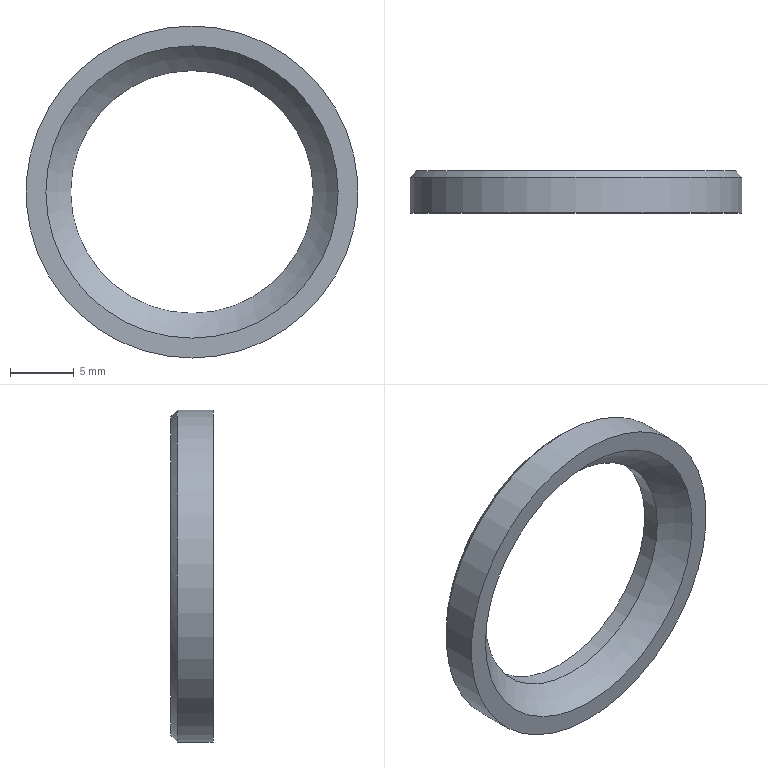Component | NX | SEAL_RING | 1 solid | 6 faces | box 26 x 3.3 x 26 mm | volume 681 mm3 | plane 2 | cylinder 2 | sphere 1 | cone 1 | commonest cylinder face diameters 19 x1 26 x1
STEP:
#1=CARTESIAN_POINT('',(0.,0.,0.));
#2=DIRECTION('',(0.,0.,1.));
#3=DIRECTION('',(1.,0.,0.));
#4=AXIS2_PLACEMENT_3D('',#1,#2,#3);
#5=CARTESIAN_POINT('',(0.,27.432,31.5));
#6=VERTEX_POINT('',#5);
#7=CARTESIAN_POINT('',(0.,27.432,19.));
#8=DIRECTION('',(0.,1.,0.));
#9=DIRECTION('',(0.,0.,1.));
#10=AXIS2_PLACEMENT_3D('',#7,#8,#9);
#11=CIRCLE('',#10,12.5);
#12=CARTESIAN_POINT('',(0.,27.432,32.));
#13=DIRECTION('',(0.,-1.,0.));
#14=DIRECTION('',(0.,0.,1.));
#15=AXIS2_PLACEMENT_3D('',#12,#13,#14);
#16=PLANE('',#15);
#17=CARTESIAN_POINT('',(-0.5,0.));
#18=CARTESIAN_POINT('',(-0.5,-21.651));
#19=CARTESIAN_POINT('',(-19.25,-10.825));
#20=CARTESIAN_POINT('',(-38.,-0.));
#21=CARTESIAN_POINT('',(-19.25,10.825));
#22=CARTESIAN_POINT('',(-0.5,21.651));
#23=CARTESIAN_POINT('',(-0.5,0.));
#24=(BOUNDED_CURVE()B_SPLINE_CURVE(2,(#17,#18,#19,#20,#21,#22,#23),.UNSPECIFIED.,.T.,.F.)B_SPLINE_CURVE_WITH_KNOTS((1,2,2,2,2,1),(-2.094,0.,2.094,4.189,6.283,8.378),.UNSPECIFIED.)CURVE()GEOMETRIC_REPRESENTATION_ITEM()RATIONAL_B_SPLINE_CURVE((1.,0.5,1.,0.5,1.,0.5,1.))REPRESENTATION_ITEM(''));
#25=(GEOMETRIC_REPRESENTATION_CONTEXT(2)PARAMETRIC_REPRESENTATION_CONTEXT()REPRESENTATION_CONTEXT('',''));
#26=DEFINITIONAL_REPRESENTATION('',(#24),#25);
#27=PCURVE('',#16,#26);
#28=CARTESIAN_POINT('',(0.,27.432,19.));
#29=DIRECTION('',(0.,-1.,0.));
#30=DIRECTION('',(0.,0.,1.));
#31=AXIS2_PLACEMENT_3D('',#28,#29,#30);
#32=CONICAL_SURFACE('',#31,12.5,0.7854);
#33=CARTESIAN_POINT('',(6.283,0.));
#34=DIRECTION('',(-1.,0.));
#35=VECTOR('',#34,1.);
#36=LINE('',#33,#35);
#37=(GEOMETRIC_REPRESENTATION_CONTEXT(2)PARAMETRIC_REPRESENTATION_CONTEXT()REPRESENTATION_CONTEXT('',''));
#38=DEFINITIONAL_REPRESENTATION('',(#36),#37);
#39=PCURVE('',#32,#38);
#40=SURFACE_CURVE('',#11,(#27,#39),.PCURVE_S1.);
#41=EDGE_CURVE('',#6,#6,#40,.T.);
#42=ORIENTED_EDGE('',*,*,#41,.T.);
#43=EDGE_LOOP('',(#42));
#44=FACE_BOUND('',#43,.T.);
#45=CARTESIAN_POINT('',(0.,27.432,9.5));
#46=VERTEX_POINT('',#45);
#47=CARTESIAN_POINT('',(0.,27.432,19.));
#48=DIRECTION('',(0.,1.,0.));
#49=DIRECTION('',(0.,0.,-1.));
#50=AXIS2_PLACEMENT_3D('',#47,#48,#49);
#51=CIRCLE('',#50,9.5);
#52=CARTESIAN_POINT('',(-22.5,0.));
#53=CARTESIAN_POINT('',(-22.5,16.454));
#54=CARTESIAN_POINT('',(-8.25,8.227));
#55=CARTESIAN_POINT('',(6.,0.));
#56=CARTESIAN_POINT('',(-8.25,-8.227));
#57=CARTESIAN_POINT('',(-22.5,-16.454));
#58=CARTESIAN_POINT('',(-22.5,0.));
#59=(BOUNDED_CURVE()B_SPLINE_CURVE(2,(#52,#53,#54,#55,#56,#57,#58),.UNSPECIFIED.,.T.,.F.)B_SPLINE_CURVE_WITH_KNOTS((1,2,2,2,2,1),(-2.094,0.,2.094,4.189,6.283,8.378),.UNSPECIFIED.)CURVE()GEOMETRIC_REPRESENTATION_ITEM()RATIONAL_B_SPLINE_CURVE((1.,0.5,1.,0.5,1.,0.5,1.))REPRESENTATION_ITEM(''));
#60=(GEOMETRIC_REPRESENTATION_CONTEXT(2)PARAMETRIC_REPRESENTATION_CONTEXT()REPRESENTATION_CONTEXT('',''));
#61=DEFINITIONAL_REPRESENTATION('',(#59),#60);
#62=PCURVE('',#16,#61);
#63=CARTESIAN_POINT('',(0.,27.432,19.));
#64=DIRECTION('',(0.,1.,0.));
#65=DIRECTION('',(0.,0.,-1.));
#66=AXIS2_PLACEMENT_3D('',#63,#64,#65);
#67=CYLINDRICAL_SURFACE('',#66,9.5);
#68=CARTESIAN_POINT('',(0.,0.));
#69=DIRECTION('',(1.,0.));
#70=VECTOR('',#69,1.);
#71=LINE('',#68,#70);
#72=(GEOMETRIC_REPRESENTATION_CONTEXT(2)PARAMETRIC_REPRESENTATION_CONTEXT()REPRESENTATION_CONTEXT('',''));
#73=DEFINITIONAL_REPRESENTATION('',(#71),#72);
#74=PCURVE('',#67,#73);
#75=SURFACE_CURVE('',#51,(#62,#74),.PCURVE_S1.);
#76=EDGE_CURVE('',#46,#46,#75,.T.);
#77=ORIENTED_EDGE('',*,*,#76,.F.);
#78=EDGE_LOOP('',(#77));
#79=FACE_BOUND('',#78,.T.);
#80=ADVANCED_FACE('',(#44,#79),#16,.F.);
#81=CARTESIAN_POINT('',(0.,26.04,9.5));
#82=VERTEX_POINT('',#81);
#83=CARTESIAN_POINT('',(0.,26.04,19.));
#84=DIRECTION('',(0.,1.,0.));
#85=DIRECTION('',(0.,0.,-1.));
#86=AXIS2_PLACEMENT_3D('',#83,#84,#85);
#87=CIRCLE('',#86,9.5);
#88=CARTESIAN_POINT('',(0.,-1.392));
#89=DIRECTION('',(1.,0.));
#90=VECTOR('',#89,1.);
#91=LINE('',#88,#90);
#92=(GEOMETRIC_REPRESENTATION_CONTEXT(2)PARAMETRIC_REPRESENTATION_CONTEXT()REPRESENTATION_CONTEXT('',''));
#93=DEFINITIONAL_REPRESENTATION('',(#91),#92);
#94=PCURVE('',#67,#93);
#95=CARTESIAN_POINT('',(0.,14.432,19.));
#96=DIRECTION('',(0.,1.,0.));
#97=DIRECTION('',(0.,0.,1.));
#98=AXIS2_PLACEMENT_3D('',#95,#96,#97);
#99=SPHERICAL_SURFACE('',#98,15.);
#100=CARTESIAN_POINT('',(3.142,0.8849));
#101=CARTESIAN_POINT('',(3.237,0.8849));
#102=CARTESIAN_POINT('',(3.427,0.8849));
#103=CARTESIAN_POINT('',(3.713,0.8849));
#104=CARTESIAN_POINT('',(3.998,0.8849));
#105=CARTESIAN_POINT('',(4.284,0.8849));
#106=CARTESIAN_POINT('',(4.57,0.8849));
#107=CARTESIAN_POINT('',(4.855,0.8849));
#108=CARTESIAN_POINT('',(5.141,0.8849));
#109=CARTESIAN_POINT('',(5.426,0.8849));
#110=CARTESIAN_POINT('',(5.712,0.8849));
#111=CARTESIAN_POINT('',(5.998,0.8849));
#112=CARTESIAN_POINT('',(6.283,0.8849));
#113=CARTESIAN_POINT('',(6.569,0.8849));
#114=CARTESIAN_POINT('',(6.854,0.8849));
#115=CARTESIAN_POINT('',(7.14,0.8849));
#116=CARTESIAN_POINT('',(7.426,0.8849));
#117=CARTESIAN_POINT('',(7.711,0.8849));
#118=CARTESIAN_POINT('',(7.997,0.8849));
#119=CARTESIAN_POINT('',(8.282,0.8849));
#120=CARTESIAN_POINT('',(8.568,0.8849));
#121=CARTESIAN_POINT('',(8.854,0.8849));
#122=CARTESIAN_POINT('',(9.139,0.8849));
#123=CARTESIAN_POINT('',(9.33,0.8849));
#124=CARTESIAN_POINT('',(9.425,0.8849));
#125=B_SPLINE_CURVE_WITH_KNOTS('',3,(#100,#101,#102,#103,#104,#105,#106,#107,#108,#109,#110,#111,#112,#113,#114,#115,#116,#117,#118,#119,#120,#121,#122,#123,#124),.UNSPECIFIED.,.F.,.F.,(4,1,1,1,1,1,1,1,1,1,1,1,1,1,1,1,1,1,1,1,1,1,4),(0.,0.2856,0.5712,0.8568,1.142,1.428,1.714,1.999,2.285,2.57,2.856,3.142,3.427,3.713,3.998,4.284,4.57,4.855,5.141,5.426,5.712,5.998,6.283),.QUASI_UNIFORM_KNOTS.);
#126=(GEOMETRIC_REPRESENTATION_CONTEXT(2)PARAMETRIC_REPRESENTATION_CONTEXT()REPRESENTATION_CONTEXT('',''));
#127=DEFINITIONAL_REPRESENTATION('',(#125),#126);
#128=PCURVE('',#99,#127);
#129=SURFACE_CURVE('',#87,(#94,#128),.PCURVE_S1.);
#130=EDGE_CURVE('',#82,#82,#129,.T.);
#131=ORIENTED_EDGE('',*,*,#130,.T.);
#132=CARTESIAN_POINT('',(0.,26.04,9.5));
#133=CARTESIAN_POINT('',(0.,27.432,9.5));
#134=B_SPLINE_CURVE_WITH_KNOTS('',1,(#132,#133),.UNSPECIFIED.,.F.,.F.,(2,2),(-1.392,0.),.PIECEWISE_BEZIER_KNOTS.);
#135=CARTESIAN_POINT('',(6.283,0.));
#136=DIRECTION('',(0.,1.));
#137=VECTOR('',#136,1.);
#138=LINE('',#135,#137);
#139=(GEOMETRIC_REPRESENTATION_CONTEXT(2)PARAMETRIC_REPRESENTATION_CONTEXT()REPRESENTATION_CONTEXT('',''));
#140=DEFINITIONAL_REPRESENTATION('',(#138),#139);
#141=PCURVE('',#67,#140);
#142=CARTESIAN_POINT('',(0.,0.));
#143=DIRECTION('',(0.,1.));
#144=VECTOR('',#143,1.);
#145=LINE('',#142,#144);
#146=(GEOMETRIC_REPRESENTATION_CONTEXT(2)PARAMETRIC_REPRESENTATION_CONTEXT()REPRESENTATION_CONTEXT('',''));
#147=DEFINITIONAL_REPRESENTATION('',(#145),#146);
#148=PCURVE('',#67,#147);
#149=SEAM_CURVE('',#134,(#141,#148),.PCURVE_S1.);
#150=EDGE_CURVE('',#82,#46,#149,.T.);
#151=ORIENTED_EDGE('',*,*,#150,.T.);
#152=ORIENTED_EDGE('',*,*,#76,.F.);
#153=ORIENTED_EDGE('',*,*,#150,.F.);
#154=EDGE_LOOP('',(#131,#151,#152,#153));
#155=FACE_BOUND('',#154,.F.);
#156=ADVANCED_FACE('',(#155),#67,.F.);
#157=CARTESIAN_POINT('',(0.,24.132,7.558));
#158=VERTEX_POINT('',#157);
#159=CARTESIAN_POINT('',(0.,24.132,19.));
#160=DIRECTION('',(0.,1.,0.));
#161=DIRECTION('',(0.,0.,-1.));
#162=AXIS2_PLACEMENT_3D('',#159,#160,#161);
#163=CIRCLE('',#162,11.442);
#164=CARTESIAN_POINT('',(3.142,0.7032));
#165=CARTESIAN_POINT('',(3.237,0.7032));
#166=CARTESIAN_POINT('',(3.427,0.7032));
#167=CARTESIAN_POINT('',(3.713,0.7032));
#168=CARTESIAN_POINT('',(3.998,0.7032));
#169=CARTESIAN_POINT('',(4.284,0.7032));
#170=CARTESIAN_POINT('',(4.57,0.7032));
#171=CARTESIAN_POINT('',(4.855,0.7032));
#172=CARTESIAN_POINT('',(5.141,0.7032));
#173=CARTESIAN_POINT('',(5.426,0.7032));
#174=CARTESIAN_POINT('',(5.712,0.7032));
#175=CARTESIAN_POINT('',(5.998,0.7032));
#176=CARTESIAN_POINT('',(6.283,0.7032));
#177=CARTESIAN_POINT('',(6.569,0.7032));
#178=CARTESIAN_POINT('',(6.854,0.7032));
#179=CARTESIAN_POINT('',(7.14,0.7032));
#180=CARTESIAN_POINT('',(7.426,0.7032));
#181=CARTESIAN_POINT('',(7.711,0.7032));
#182=CARTESIAN_POINT('',(7.997,0.7032));
#183=CARTESIAN_POINT('',(8.282,0.7032));
#184=CARTESIAN_POINT('',(8.568,0.7032));
#185=CARTESIAN_POINT('',(8.854,0.7032));
#186=CARTESIAN_POINT('',(9.139,0.7032));
#187=CARTESIAN_POINT('',(9.33,0.7032));
#188=CARTESIAN_POINT('',(9.425,0.7032));
#189=B_SPLINE_CURVE_WITH_KNOTS('',3,(#164,#165,#166,#167,#168,#169,#170,#171,#172,#173,#174,#175,#176,#177,#178,#179,#180,#181,#182,#183,#184,#185,#186,#187,#188),.UNSPECIFIED.,.F.,.F.,(4,1,1,1,1,1,1,1,1,1,1,1,1,1,1,1,1,1,1,1,1,1,4),(0.,0.2856,0.5712,0.8568,1.142,1.428,1.714,1.999,2.285,2.57,2.856,3.142,3.427,3.713,3.998,4.284,4.57,4.855,5.141,5.426,5.712,5.998,6.283),.QUASI_UNIFORM_KNOTS.);
#190=(GEOMETRIC_REPRESENTATION_CONTEXT(2)PARAMETRIC_REPRESENTATION_CONTEXT()REPRESENTATION_CONTEXT('',''));
#191=DEFINITIONAL_REPRESENTATION('',(#189),#190);
#192=PCURVE('',#99,#191);
#193=CARTESIAN_POINT('',(0.,24.132,30.442));
#194=DIRECTION('',(0.,1.,0.));
#195=DIRECTION('',(0.,0.,-1.));
#196=AXIS2_PLACEMENT_3D('',#193,#194,#195);
#197=PLANE('',#196);
#198=CARTESIAN_POINT('',(11.442,0.));
#199=DIRECTION('',(1.,0.));
#200=AXIS2_PLACEMENT_2D('',#198,#199);
#201=CIRCLE('',#200,11.442);
#202=(GEOMETRIC_REPRESENTATION_CONTEXT(2)PARAMETRIC_REPRESENTATION_CONTEXT()REPRESENTATION_CONTEXT('',''));
#203=DEFINITIONAL_REPRESENTATION('',(#201),#202);
#204=PCURVE('',#197,#203);
#205=SURFACE_CURVE('',#163,(#192,#204),.PCURVE_S1.);
#206=EDGE_CURVE('',#158,#158,#205,.T.);
#207=ORIENTED_EDGE('',*,*,#206,.T.);
#208=CARTESIAN_POINT('',(0.,24.132,7.558));
#209=CARTESIAN_POINT('',(0.,24.652,7.999));
#210=CARTESIAN_POINT('',(0.,25.145,8.471));
#211=CARTESIAN_POINT('',(0.,25.609,8.973));
#212=CARTESIAN_POINT('',(0.,26.04,9.5));
#213=B_SPLINE_CURVE_WITH_KNOTS('',4,(#208,#209,#210,#211,#212),.UNSPECIFIED.,.F.,.F.,(5,5),(0.7032,0.8849),.PIECEWISE_BEZIER_KNOTS.);
#214=CARTESIAN_POINT('',(9.425,0.));
#215=DIRECTION('',(0.,1.));
#216=VECTOR('',#215,1.);
#217=LINE('',#214,#216);
#218=(GEOMETRIC_REPRESENTATION_CONTEXT(2)PARAMETRIC_REPRESENTATION_CONTEXT()REPRESENTATION_CONTEXT('',''));
#219=DEFINITIONAL_REPRESENTATION('',(#217),#218);
#220=PCURVE('',#99,#219);
#221=CARTESIAN_POINT('',(3.142,0.));
#222=DIRECTION('',(0.,1.));
#223=VECTOR('',#222,1.);
#224=LINE('',#221,#223);
#225=(GEOMETRIC_REPRESENTATION_CONTEXT(2)PARAMETRIC_REPRESENTATION_CONTEXT()REPRESENTATION_CONTEXT('',''));
#226=DEFINITIONAL_REPRESENTATION('',(#224),#225);
#227=PCURVE('',#99,#226);
#228=SEAM_CURVE('',#213,(#220,#227),.PCURVE_S1.);
#229=EDGE_CURVE('',#158,#82,#228,.T.);
#230=ORIENTED_EDGE('',*,*,#229,.T.);
#231=ORIENTED_EDGE('',*,*,#130,.F.);
#232=ORIENTED_EDGE('',*,*,#229,.F.);
#233=EDGE_LOOP('',(#207,#230,#231,#232));
#234=FACE_BOUND('',#233,.F.);
#235=ADVANCED_FACE('',(#234),#99,.F.);
#236=CARTESIAN_POINT('',(0.,24.132,6.));
#237=VERTEX_POINT('',#236);
#238=CARTESIAN_POINT('',(0.,24.132,19.));
#239=DIRECTION('',(0.,1.,0.));
#240=DIRECTION('',(0.,0.,-1.));
#241=AXIS2_PLACEMENT_3D('',#238,#239,#240);
#242=CIRCLE('',#241,13.);
#243=CARTESIAN_POINT('',(11.442,0.));
#244=DIRECTION('',(1.,0.));
#245=AXIS2_PLACEMENT_2D('',#243,#244);
#246=CIRCLE('',#245,13.);
#247=(GEOMETRIC_REPRESENTATION_CONTEXT(2)PARAMETRIC_REPRESENTATION_CONTEXT()REPRESENTATION_CONTEXT('',''));
#248=DEFINITIONAL_REPRESENTATION('',(#246),#247);
#249=PCURVE('',#197,#248);
#250=CARTESIAN_POINT('',(0.,27.432,19.));
#251=DIRECTION('',(0.,1.,0.));
#252=DIRECTION('',(0.,0.,-1.));
#253=AXIS2_PLACEMENT_3D('',#250,#251,#252);
#254=CYLINDRICAL_SURFACE('',#253,13.);
#255=CARTESIAN_POINT('',(0.,-3.3));
#256=DIRECTION('',(1.,0.));
#257=VECTOR('',#256,1.);
#258=LINE('',#255,#257);
#259=(GEOMETRIC_REPRESENTATION_CONTEXT(2)PARAMETRIC_REPRESENTATION_CONTEXT()REPRESENTATION_CONTEXT('',''));
#260=DEFINITIONAL_REPRESENTATION('',(#258),#259);
#261=PCURVE('',#254,#260);
#262=SURFACE_CURVE('',#242,(#249,#261),.PCURVE_S1.);
#263=EDGE_CURVE('',#237,#237,#262,.T.);
#264=ORIENTED_EDGE('',*,*,#263,.F.);
#265=EDGE_LOOP('',(#264));
#266=FACE_BOUND('',#265,.T.);
#267=ORIENTED_EDGE('',*,*,#206,.T.);
#268=EDGE_LOOP('',(#267));
#269=FACE_BOUND('',#268,.T.);
#270=ADVANCED_FACE('',(#266,#269),#197,.F.);
#271=CARTESIAN_POINT('',(0.,26.932,32.));
#272=VERTEX_POINT('',#271);
#273=CARTESIAN_POINT('',(0.,26.932,6.));
#274=VERTEX_POINT('',#273);
#275=CARTESIAN_POINT('',(0.,26.932,19.));
#276=DIRECTION('',(0.,-1.,0.));
#277=DIRECTION('',(0.,0.,1.));
#278=AXIS2_PLACEMENT_3D('',#275,#276,#277);
#279=CIRCLE('',#278,13.);
#280=CARTESIAN_POINT('',(3.142,-0.5));
#281=DIRECTION('',(-1.,0.));
#282=VECTOR('',#281,1.);
#283=LINE('',#280,#282);
#284=(GEOMETRIC_REPRESENTATION_CONTEXT(2)PARAMETRIC_REPRESENTATION_CONTEXT()REPRESENTATION_CONTEXT('',''));
#285=DEFINITIONAL_REPRESENTATION('',(#283),#284);
#286=PCURVE('',#254,#285);
#287=CARTESIAN_POINT('',(0.,0.5));
#288=DIRECTION('',(1.,0.));
#289=VECTOR('',#288,1.);
#290=LINE('',#287,#289);
#291=(GEOMETRIC_REPRESENTATION_CONTEXT(2)PARAMETRIC_REPRESENTATION_CONTEXT()REPRESENTATION_CONTEXT('',''));
#292=DEFINITIONAL_REPRESENTATION('',(#290),#291);
#293=PCURVE('',#32,#292);
#294=SURFACE_CURVE('',#279,(#286,#293),.PCURVE_S1.);
#295=EDGE_CURVE('',#272,#274,#294,.T.);
#296=ORIENTED_EDGE('',*,*,#295,.T.);
#297=CARTESIAN_POINT('',(0.,24.132,6.));
#298=CARTESIAN_POINT('',(0.,26.932,6.));
#299=B_SPLINE_CURVE_WITH_KNOTS('',1,(#297,#298),.UNSPECIFIED.,.F.,.F.,(2,2),(-3.3,-0.5),.PIECEWISE_BEZIER_KNOTS.);
#300=CARTESIAN_POINT('',(0.,0.));
#301=DIRECTION('',(0.,1.));
#302=VECTOR('',#301,1.);
#303=LINE('',#300,#302);
#304=(GEOMETRIC_REPRESENTATION_CONTEXT(2)PARAMETRIC_REPRESENTATION_CONTEXT()REPRESENTATION_CONTEXT('',''));
#305=DEFINITIONAL_REPRESENTATION('',(#303),#304);
#306=PCURVE('',#254,#305);
#307=CARTESIAN_POINT('',(6.283,0.));
#308=DIRECTION('',(0.,1.));
#309=VECTOR('',#308,1.);
#310=LINE('',#307,#309);
#311=(GEOMETRIC_REPRESENTATION_CONTEXT(2)PARAMETRIC_REPRESENTATION_CONTEXT()REPRESENTATION_CONTEXT('',''));
#312=DEFINITIONAL_REPRESENTATION('',(#310),#311);
#313=PCURVE('',#254,#312);
#314=SEAM_CURVE('',#299,(#306,#313),.PCURVE_S1.);
#315=EDGE_CURVE('',#237,#274,#314,.T.);
#316=ORIENTED_EDGE('',*,*,#315,.F.);
#317=ORIENTED_EDGE('',*,*,#263,.T.);
#318=ORIENTED_EDGE('',*,*,#315,.T.);
#319=CARTESIAN_POINT('',(0.,26.932,19.));
#320=DIRECTION('',(0.,-1.,0.));
#321=DIRECTION('',(0.,0.,1.));
#322=AXIS2_PLACEMENT_3D('',#319,#320,#321);
#323=CIRCLE('',#322,13.);
#324=CARTESIAN_POINT('',(9.425,-0.5));
#325=DIRECTION('',(-1.,0.));
#326=VECTOR('',#325,1.);
#327=LINE('',#324,#326);
#328=(GEOMETRIC_REPRESENTATION_CONTEXT(2)PARAMETRIC_REPRESENTATION_CONTEXT()REPRESENTATION_CONTEXT('',''));
#329=DEFINITIONAL_REPRESENTATION('',(#327),#328);
#330=PCURVE('',#254,#329);
#331=CARTESIAN_POINT('',(0.,0.5));
#332=DIRECTION('',(1.,0.));
#333=VECTOR('',#332,1.);
#334=LINE('',#331,#333);
#335=(GEOMETRIC_REPRESENTATION_CONTEXT(2)PARAMETRIC_REPRESENTATION_CONTEXT()REPRESENTATION_CONTEXT('',''));
#336=DEFINITIONAL_REPRESENTATION('',(#334),#335);
#337=PCURVE('',#32,#336);
#338=SURFACE_CURVE('',#323,(#330,#337),.PCURVE_S1.);
#339=EDGE_CURVE('',#274,#272,#338,.T.);
#340=ORIENTED_EDGE('',*,*,#339,.T.);
#341=EDGE_LOOP('',(#296,#316,#317,#318,#340));
#342=FACE_BOUND('',#341,.T.);
#343=ADVANCED_FACE('',(#342),#254,.T.);
#344=ORIENTED_EDGE('',*,*,#295,.F.);
#345=CARTESIAN_POINT('',(0.,27.432,31.5));
#346=CARTESIAN_POINT('',(0.,26.932,32.));
#347=B_SPLINE_CURVE_WITH_KNOTS('',1,(#345,#346),.UNSPECIFIED.,.F.,.F.,(2,2),(0.,0.7071),.PIECEWISE_BEZIER_KNOTS.);
#348=CARTESIAN_POINT('',(0.,0.));
#349=DIRECTION('',(0.,1.));
#350=VECTOR('',#349,1.);
#351=LINE('',#348,#350);
#352=(GEOMETRIC_REPRESENTATION_CONTEXT(2)PARAMETRIC_REPRESENTATION_CONTEXT()REPRESENTATION_CONTEXT('',''));
#353=DEFINITIONAL_REPRESENTATION('',(#351),#352);
#354=PCURVE('',#32,#353);
#355=CARTESIAN_POINT('',(6.283,0.));
#356=DIRECTION('',(0.,1.));
#357=VECTOR('',#356,1.);
#358=LINE('',#355,#357);
#359=(GEOMETRIC_REPRESENTATION_CONTEXT(2)PARAMETRIC_REPRESENTATION_CONTEXT()REPRESENTATION_CONTEXT('',''));
#360=DEFINITIONAL_REPRESENTATION('',(#358),#359);
#361=PCURVE('',#32,#360);
#362=SEAM_CURVE('',#347,(#354,#361),.PCURVE_S1.);
#363=EDGE_CURVE('',#6,#272,#362,.T.);
#364=ORIENTED_EDGE('',*,*,#363,.F.);
#365=ORIENTED_EDGE('',*,*,#41,.F.);
#366=ORIENTED_EDGE('',*,*,#363,.T.);
#367=ORIENTED_EDGE('',*,*,#339,.F.);
#368=EDGE_LOOP('',(#344,#364,#365,#366,#367));
#369=FACE_BOUND('',#368,.T.);
#370=ADVANCED_FACE('',(#369),#32,.T.);
#371=CLOSED_SHELL('',(#80,#156,#235,#270,#343,#370));
#372=MANIFOLD_SOLID_BREP('',#371);
#373=(LENGTH_UNIT()NAMED_UNIT(*)SI_UNIT(.MILLI.,.METRE.));
#374=UNCERTAINTY_MEASURE_WITH_UNIT(LENGTH_MEASURE(0.00001),#373,'','');
#375=(NAMED_UNIT(*)PLANE_ANGLE_UNIT()SI_UNIT($,.RADIAN.));
#376=(NAMED_UNIT(*)SI_UNIT($,.STERADIAN.)SOLID_ANGLE_UNIT());
#377=(GEOMETRIC_REPRESENTATION_CONTEXT(3)GLOBAL_UNCERTAINTY_ASSIGNED_CONTEXT((#374))GLOBAL_UNIT_ASSIGNED_CONTEXT((#373,#375,#376))REPRESENTATION_CONTEXT('',''));
#378=ADVANCED_BREP_SHAPE_REPRESENTATION('',(#4,#372),#377);